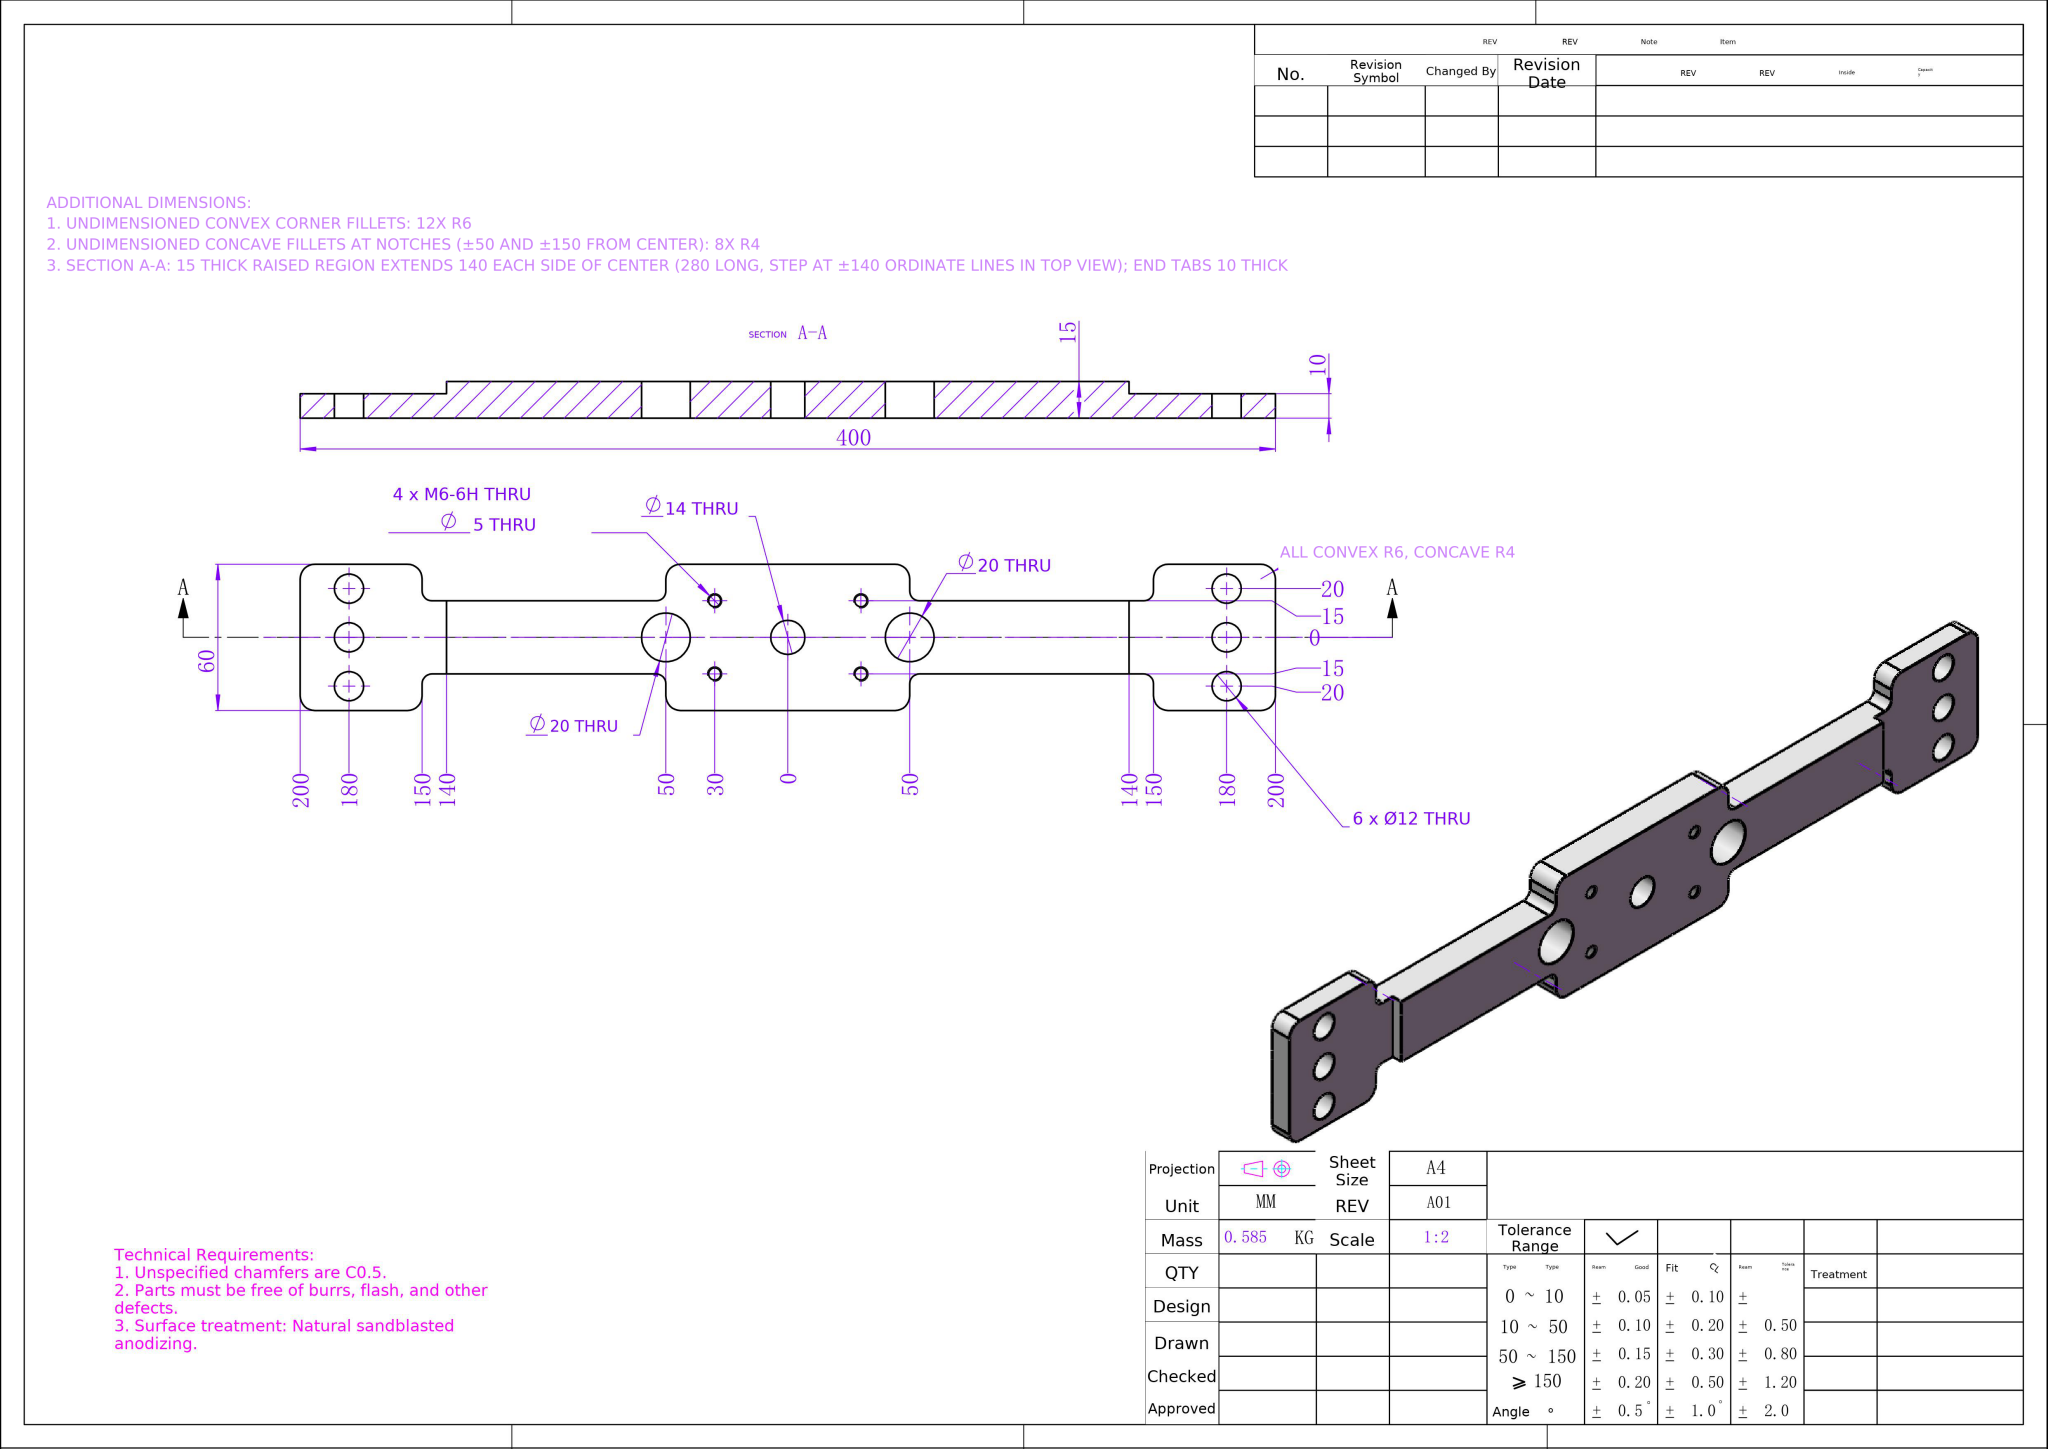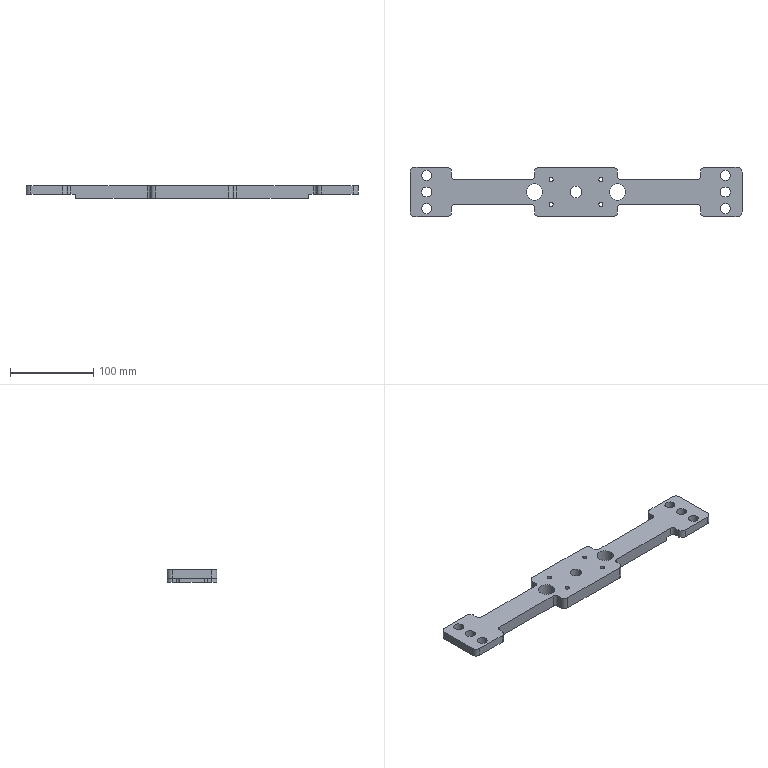Part | NX | mm | 1 solid | 72 faces | box 400 x 60 x 15 mm | volume 216564 mm3 | cylinder 46 | plane 26 | commonest cylinder face diameters 12 x24 5 x8 8 x8 20 x4 14 x2